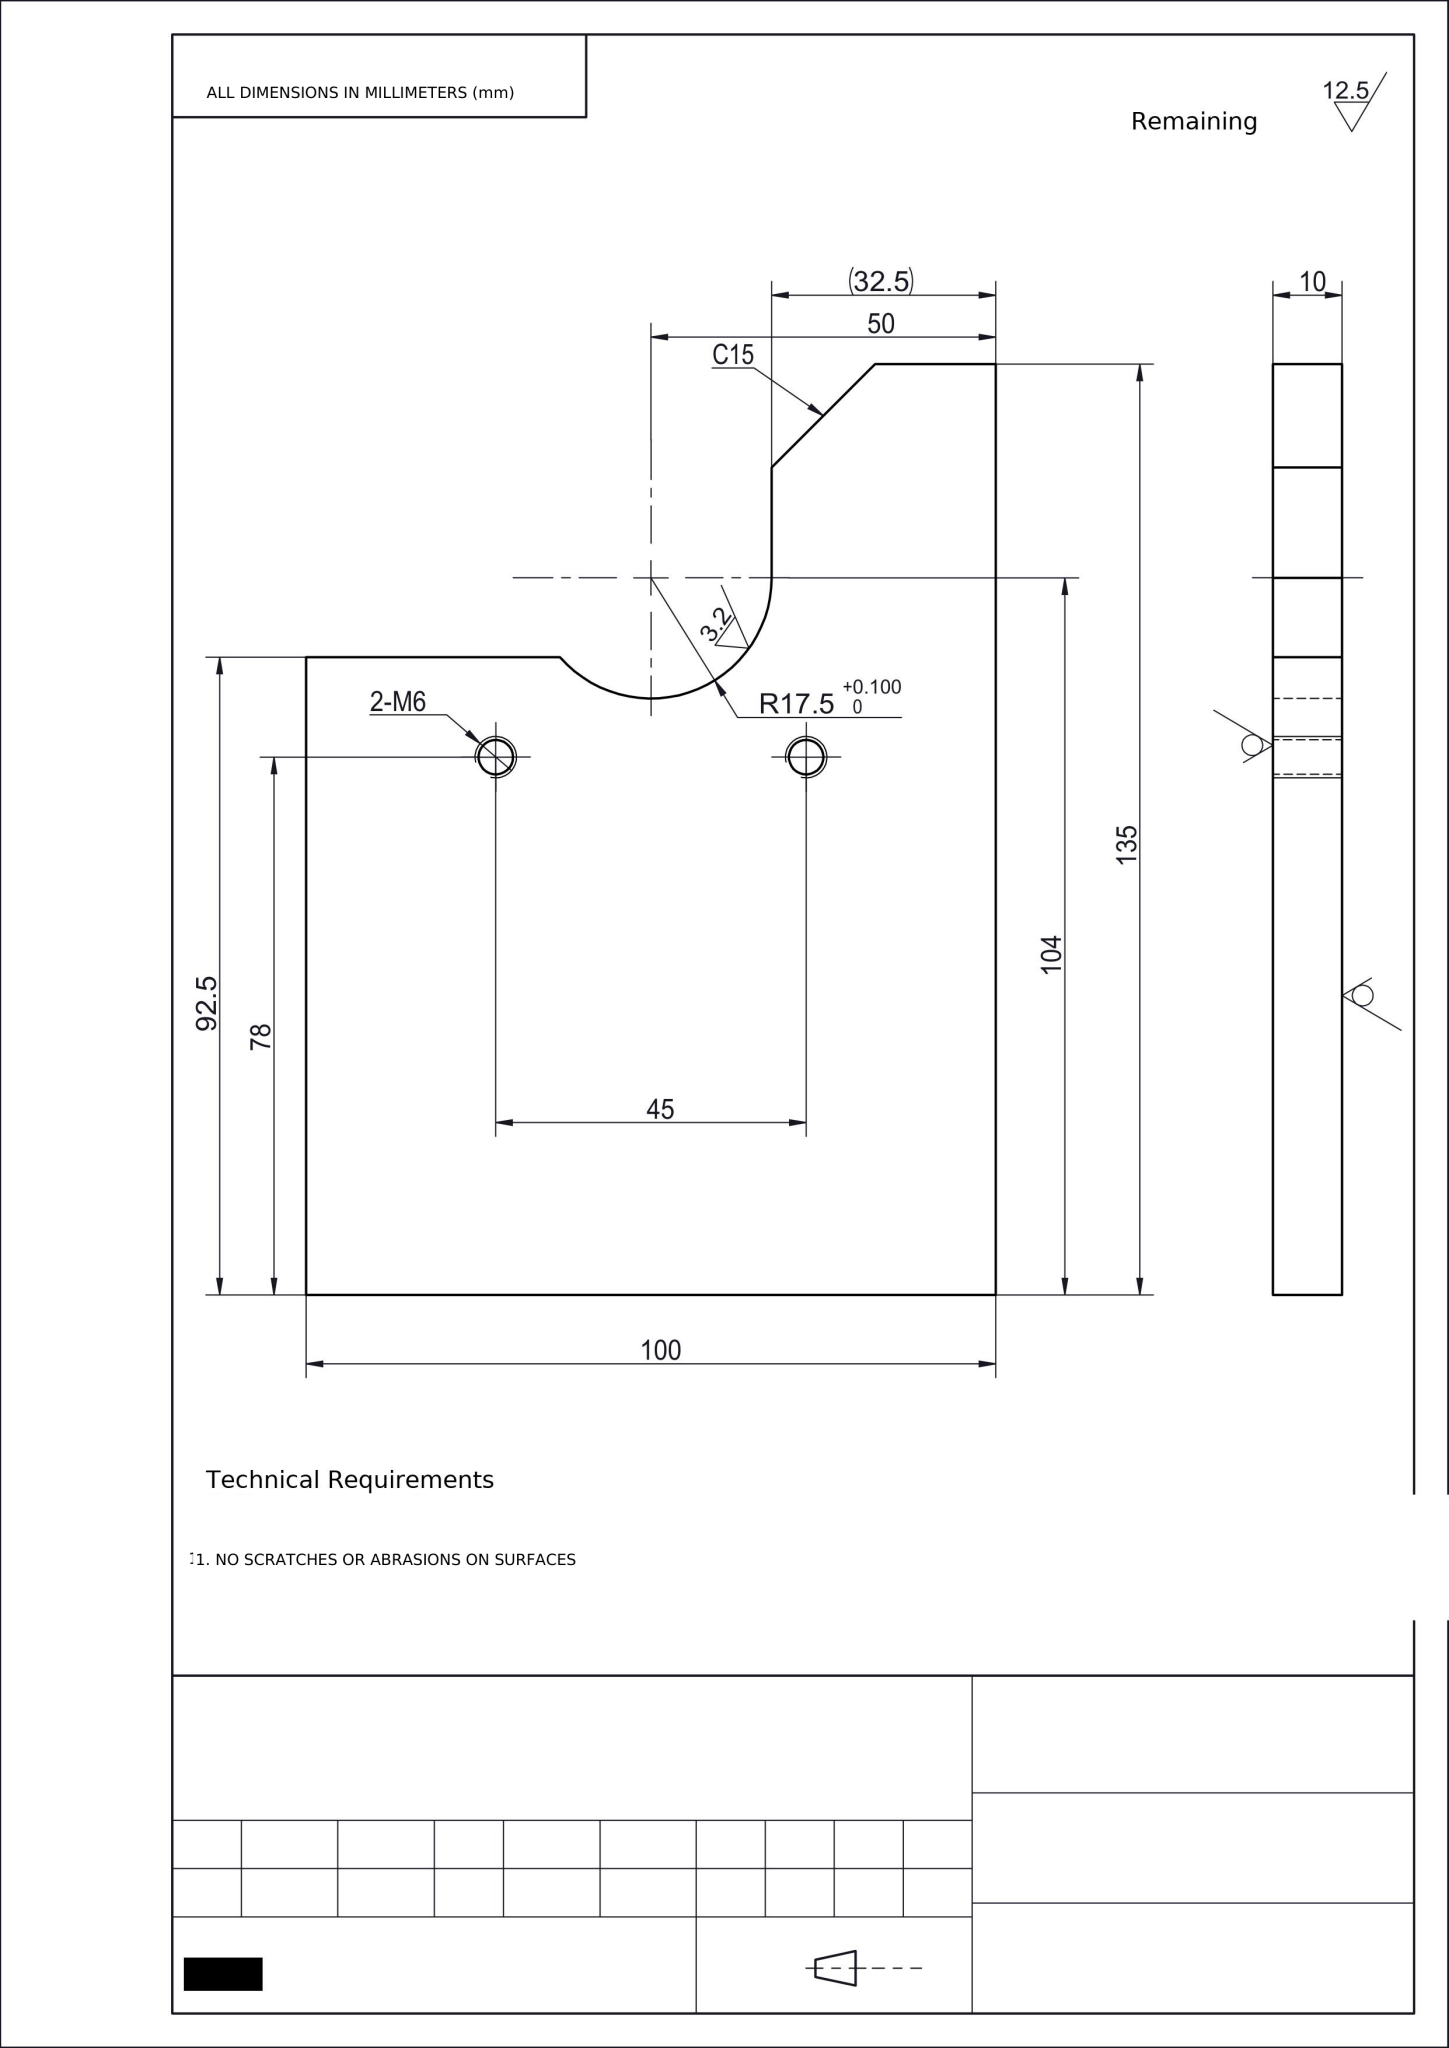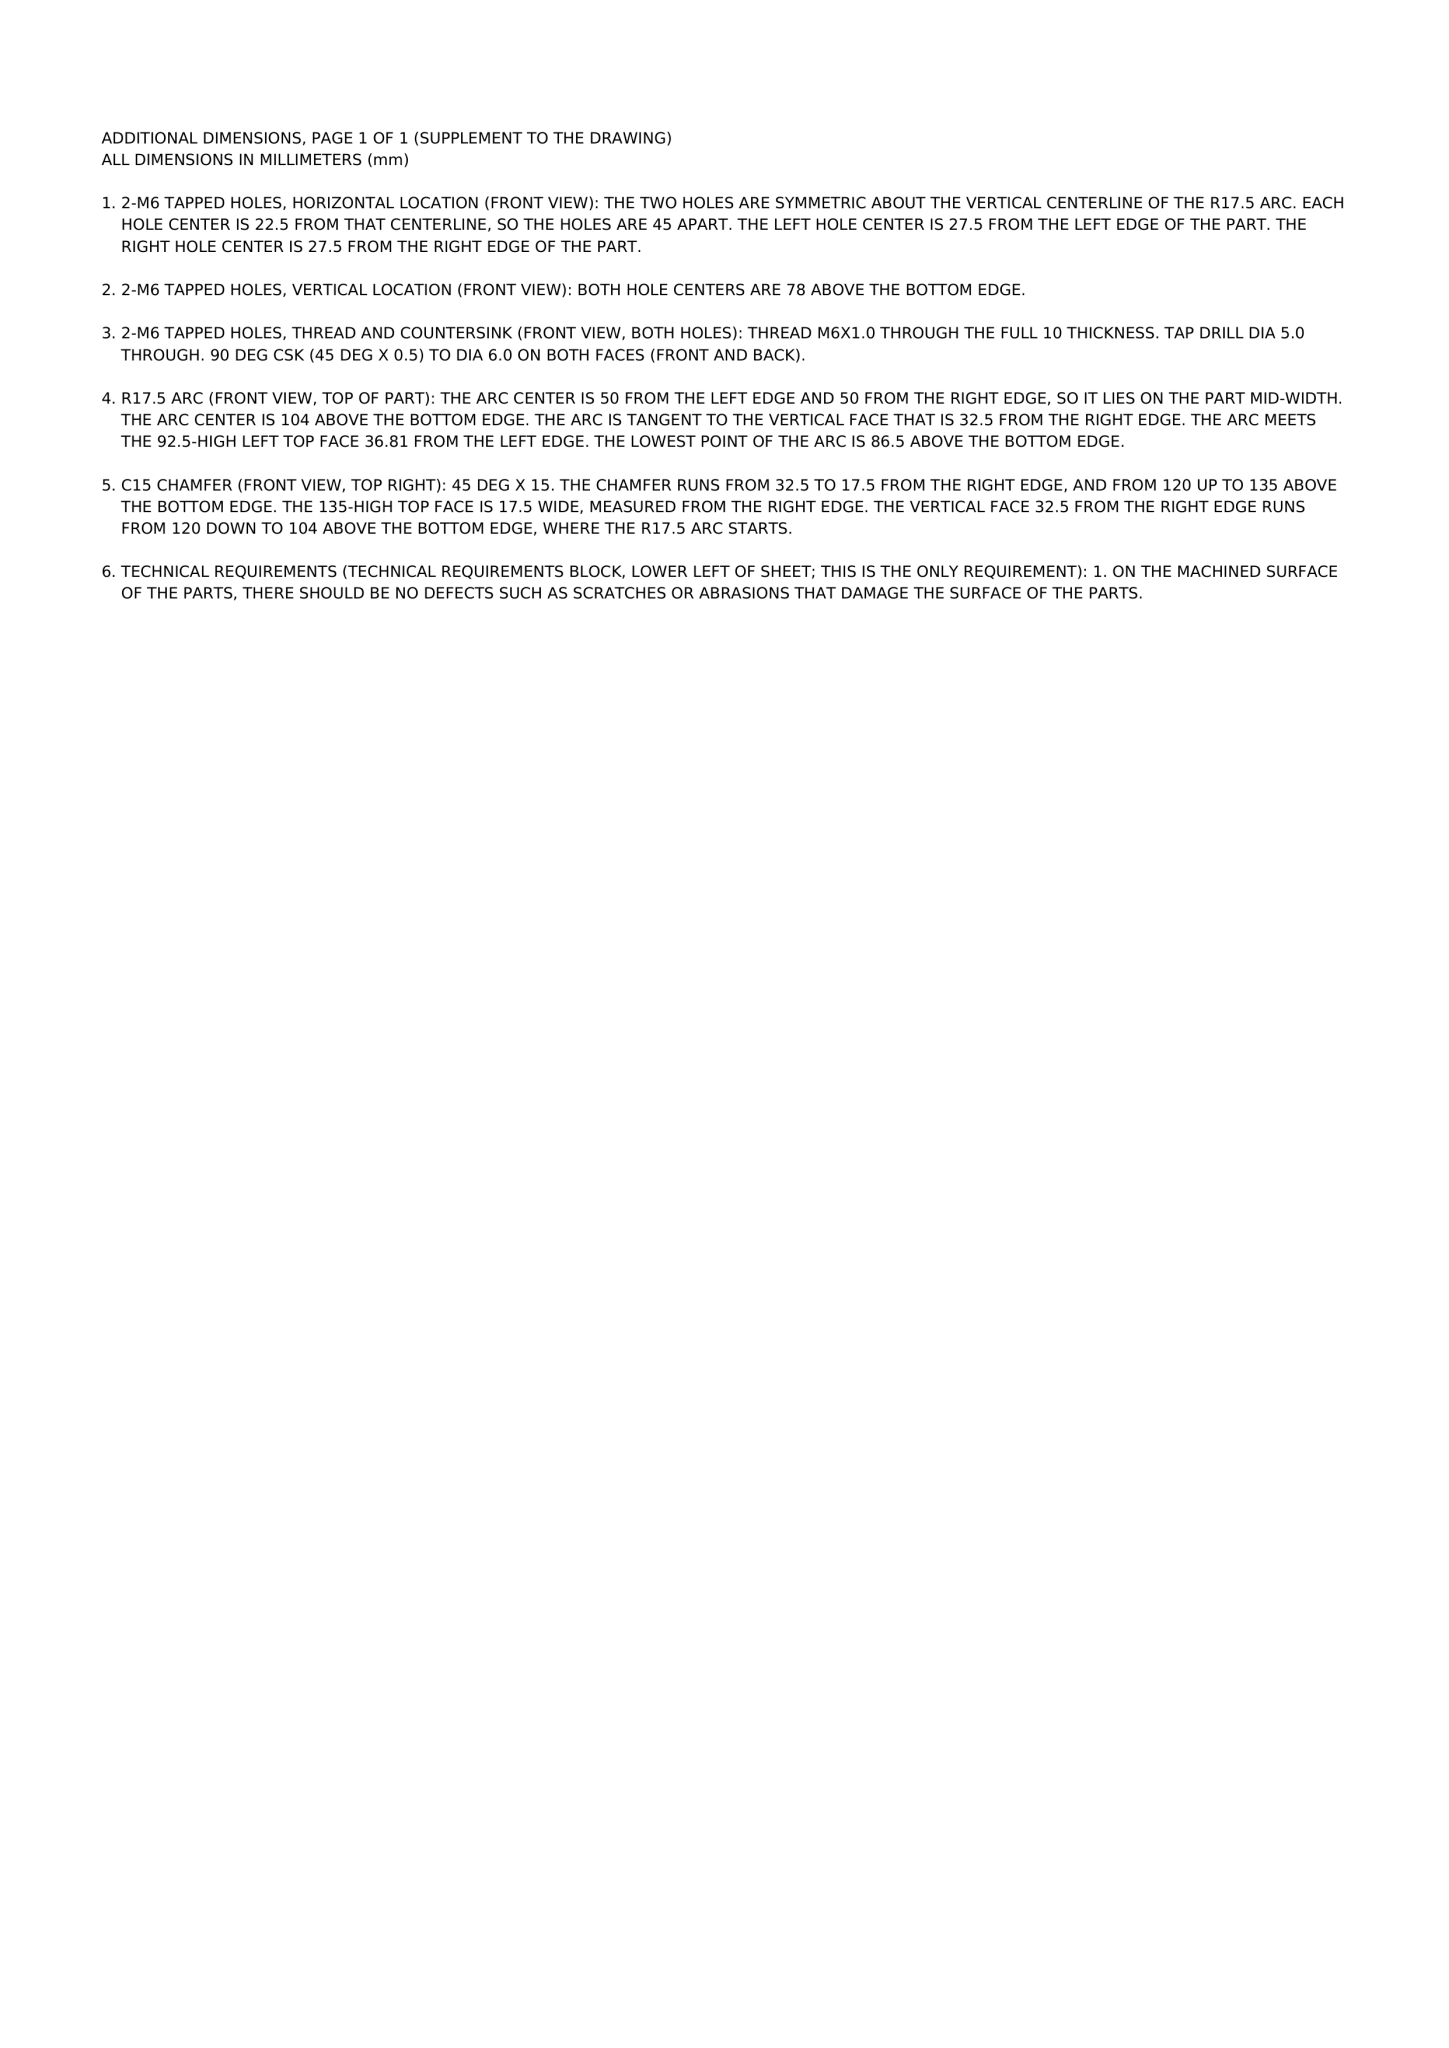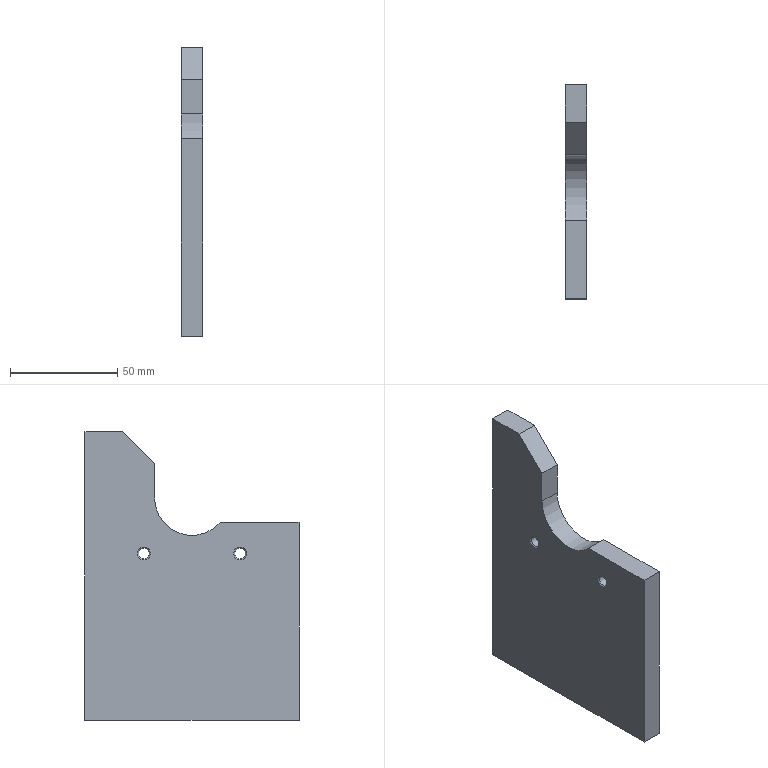Part | NX | mm | 1 solid | 16 faces | box 10 x 100 x 135 mm | volume 103845 mm3 | plane 9 | cone 4 | cylinder 3 | commonest cylinder face diameters 5 x2 35 x1
STEP:
#1=CARTESIAN_POINT('',(0.,0.,0.));
#2=DIRECTION('',(0.,0.,1.));
#3=DIRECTION('',(1.,0.,0.));
#4=AXIS2_PLACEMENT_3D('',#1,#2,#3);
#5=(LENGTH_UNIT()NAMED_UNIT(*)SI_UNIT(.MILLI.,.METRE.));
#6=UNCERTAINTY_MEASURE_WITH_UNIT(LENGTH_MEASURE(0.00002),#5,'','');
#7=(NAMED_UNIT(*)PLANE_ANGLE_UNIT()SI_UNIT($,.RADIAN.));
#8=PLANE_ANGLE_MEASURE_WITH_UNIT(PLANE_ANGLE_MEASURE(0.01745),#7);
#9=DIMENSIONAL_EXPONENTS(0.,0.,0.,0.,0.,0.,0.);
#10=(CONVERSION_BASED_UNIT('',#8)NAMED_UNIT(#9)PLANE_ANGLE_UNIT());
#11=(NAMED_UNIT(*)SI_UNIT($,.STERADIAN.)SOLID_ANGLE_UNIT());
#12=(GEOMETRIC_REPRESENTATION_CONTEXT(3)GLOBAL_UNCERTAINTY_ASSIGNED_CONTEXT((#6))GLOBAL_UNIT_ASSIGNED_CONTEXT((#5,#10,#11))REPRESENTATION_CONTEXT('',''));
#13=SHAPE_REPRESENTATION('',(#4),#12);
#14=CARTESIAN_POINT('',(0.,-50.,92.5));
#15=VERTEX_POINT('',#14);
#16=CARTESIAN_POINT('',(0.,-50.,0.));
#17=VERTEX_POINT('',#16);
#18=CARTESIAN_POINT('',(0.,-50.,92.5));
#19=DIRECTION('',(0.,0.,-1.));
#20=VECTOR('',#19,1.);
#21=LINE('',#18,#20);
#22=EDGE_CURVE('',#15,#17,#21,.T.);
#23=ORIENTED_EDGE('',*,*,#22,.T.);
#24=CARTESIAN_POINT('',(10.,-50.,0.));
#25=VERTEX_POINT('',#24);
#26=CARTESIAN_POINT('',(10.,-50.,0.));
#27=DIRECTION('',(-1.,0.,0.));
#28=VECTOR('',#27,1.);
#29=LINE('',#26,#28);
#30=EDGE_CURVE('',#25,#17,#29,.T.);
#31=ORIENTED_EDGE('',*,*,#30,.F.);
#32=CARTESIAN_POINT('',(10.,-50.,92.5));
#33=VERTEX_POINT('',#32);
#34=CARTESIAN_POINT('',(10.,-50.,92.5));
#35=DIRECTION('',(0.,0.,-1.));
#36=VECTOR('',#35,1.);
#37=LINE('',#34,#36);
#38=EDGE_CURVE('',#33,#25,#37,.T.);
#39=ORIENTED_EDGE('',*,*,#38,.F.);
#40=CARTESIAN_POINT('',(10.,-50.,92.5));
#41=DIRECTION('',(-1.,0.,0.));
#42=VECTOR('',#41,1.);
#43=LINE('',#40,#42);
#44=EDGE_CURVE('',#33,#15,#43,.T.);
#45=ORIENTED_EDGE('',*,*,#44,.T.);
#46=EDGE_LOOP('',(#23,#31,#39,#45));
#47=FACE_OUTER_BOUND('',#46,.T.);
#48=CARTESIAN_POINT('',(10.,-50.,92.5));
#49=DIRECTION('',(0.,1.,0.));
#50=DIRECTION('',(0.,0.,1.));
#51=AXIS2_PLACEMENT_3D('',#48,#49,#50);
#52=PLANE('',#51);
#53=ADVANCED_FACE('',(#47),#52,.F.);
#54=CARTESIAN_POINT('',(0.,50.,0.));
#55=VERTEX_POINT('',#54);
#56=CARTESIAN_POINT('',(0.,-50.,0.));
#57=DIRECTION('',(0.,1.,0.));
#58=VECTOR('',#57,1.);
#59=LINE('',#56,#58);
#60=EDGE_CURVE('',#17,#55,#59,.T.);
#61=ORIENTED_EDGE('',*,*,#60,.T.);
#62=CARTESIAN_POINT('',(10.,50.,0.));
#63=VERTEX_POINT('',#62);
#64=CARTESIAN_POINT('',(10.,50.,0.));
#65=DIRECTION('',(-1.,0.,0.));
#66=VECTOR('',#65,1.);
#67=LINE('',#64,#66);
#68=EDGE_CURVE('',#63,#55,#67,.T.);
#69=ORIENTED_EDGE('',*,*,#68,.F.);
#70=CARTESIAN_POINT('',(10.,-50.,0.));
#71=DIRECTION('',(0.,1.,0.));
#72=VECTOR('',#71,1.);
#73=LINE('',#70,#72);
#74=EDGE_CURVE('',#25,#63,#73,.T.);
#75=ORIENTED_EDGE('',*,*,#74,.F.);
#76=ORIENTED_EDGE('',*,*,#30,.T.);
#77=EDGE_LOOP('',(#61,#69,#75,#76));
#78=FACE_OUTER_BOUND('',#77,.T.);
#79=CARTESIAN_POINT('',(10.,-50.,0.));
#80=DIRECTION('',(0.,0.,1.));
#81=DIRECTION('',(1.,0.,0.));
#82=AXIS2_PLACEMENT_3D('',#79,#80,#81);
#83=PLANE('',#82);
#84=ADVANCED_FACE('',(#78),#83,.F.);
#85=CARTESIAN_POINT('',(0.,50.,135.));
#86=VERTEX_POINT('',#85);
#87=CARTESIAN_POINT('',(0.,50.,0.));
#88=DIRECTION('',(0.,0.,1.));
#89=VECTOR('',#88,1.);
#90=LINE('',#87,#89);
#91=EDGE_CURVE('',#55,#86,#90,.T.);
#92=ORIENTED_EDGE('',*,*,#91,.T.);
#93=CARTESIAN_POINT('',(10.,50.,135.));
#94=VERTEX_POINT('',#93);
#95=CARTESIAN_POINT('',(10.,50.,135.));
#96=DIRECTION('',(-1.,0.,0.));
#97=VECTOR('',#96,1.);
#98=LINE('',#95,#97);
#99=EDGE_CURVE('',#94,#86,#98,.T.);
#100=ORIENTED_EDGE('',*,*,#99,.F.);
#101=CARTESIAN_POINT('',(10.,50.,0.));
#102=DIRECTION('',(0.,0.,1.));
#103=VECTOR('',#102,1.);
#104=LINE('',#101,#103);
#105=EDGE_CURVE('',#63,#94,#104,.T.);
#106=ORIENTED_EDGE('',*,*,#105,.F.);
#107=ORIENTED_EDGE('',*,*,#68,.T.);
#108=EDGE_LOOP('',(#92,#100,#106,#107));
#109=FACE_OUTER_BOUND('',#108,.T.);
#110=CARTESIAN_POINT('',(10.,50.,0.));
#111=DIRECTION('',(0.,-1.,0.));
#112=DIRECTION('',(0.,0.,-1.));
#113=AXIS2_PLACEMENT_3D('',#110,#111,#112);
#114=PLANE('',#113);
#115=ADVANCED_FACE('',(#109),#114,.F.);
#116=CARTESIAN_POINT('',(0.,32.5,135.));
#117=VERTEX_POINT('',#116);
#118=CARTESIAN_POINT('',(0.,50.,135.));
#119=DIRECTION('',(0.,-1.,0.));
#120=VECTOR('',#119,1.);
#121=LINE('',#118,#120);
#122=EDGE_CURVE('',#86,#117,#121,.T.);
#123=ORIENTED_EDGE('',*,*,#122,.T.);
#124=CARTESIAN_POINT('',(10.,32.5,135.));
#125=VERTEX_POINT('',#124);
#126=CARTESIAN_POINT('',(10.,32.5,135.));
#127=DIRECTION('',(1.,0.,0.));
#128=VECTOR('',#127,1.);
#129=LINE('',#126,#128);
#130=EDGE_CURVE('',#117,#125,#129,.T.);
#131=ORIENTED_EDGE('',*,*,#130,.T.);
#132=CARTESIAN_POINT('',(10.,50.,135.));
#133=DIRECTION('',(0.,-1.,0.));
#134=VECTOR('',#133,1.);
#135=LINE('',#132,#134);
#136=EDGE_CURVE('',#94,#125,#135,.T.);
#137=ORIENTED_EDGE('',*,*,#136,.F.);
#138=ORIENTED_EDGE('',*,*,#99,.T.);
#139=EDGE_LOOP('',(#123,#131,#137,#138));
#140=FACE_OUTER_BOUND('',#139,.T.);
#141=CARTESIAN_POINT('',(10.,50.,135.));
#142=DIRECTION('',(0.,0.,-1.));
#143=DIRECTION('',(-1.,0.,0.));
#144=AXIS2_PLACEMENT_3D('',#141,#142,#143);
#145=PLANE('',#144);
#146=ADVANCED_FACE('',(#140),#145,.F.);
#147=CARTESIAN_POINT('',(10.,17.5,120.));
#148=VERTEX_POINT('',#147);
#149=CARTESIAN_POINT('',(10.,17.5,104.));
#150=VERTEX_POINT('',#149);
#151=CARTESIAN_POINT('',(10.,17.5,135.));
#152=DIRECTION('',(0.,0.,-1.));
#153=VECTOR('',#152,1.);
#154=LINE('',#151,#153);
#155=EDGE_CURVE('',#148,#150,#154,.T.);
#156=ORIENTED_EDGE('',*,*,#155,.F.);
#157=CARTESIAN_POINT('',(0.,17.5,120.));
#158=VERTEX_POINT('',#157);
#159=CARTESIAN_POINT('',(10.,17.5,120.));
#160=DIRECTION('',(-1.,0.,0.));
#161=VECTOR('',#160,1.);
#162=LINE('',#159,#161);
#163=EDGE_CURVE('',#148,#158,#162,.T.);
#164=ORIENTED_EDGE('',*,*,#163,.T.);
#165=CARTESIAN_POINT('',(0.,17.5,104.));
#166=VERTEX_POINT('',#165);
#167=CARTESIAN_POINT('',(0.,17.5,135.));
#168=DIRECTION('',(0.,0.,-1.));
#169=VECTOR('',#168,1.);
#170=LINE('',#167,#169);
#171=EDGE_CURVE('',#158,#166,#170,.T.);
#172=ORIENTED_EDGE('',*,*,#171,.T.);
#173=CARTESIAN_POINT('',(10.,17.5,104.));
#174=DIRECTION('',(-1.,0.,0.));
#175=VECTOR('',#174,1.);
#176=LINE('',#173,#175);
#177=EDGE_CURVE('',#150,#166,#176,.T.);
#178=ORIENTED_EDGE('',*,*,#177,.F.);
#179=EDGE_LOOP('',(#156,#164,#172,#178));
#180=FACE_OUTER_BOUND('',#179,.T.);
#181=CARTESIAN_POINT('',(10.,17.5,135.));
#182=DIRECTION('',(0.,1.,0.));
#183=DIRECTION('',(0.,0.,1.));
#184=AXIS2_PLACEMENT_3D('',#181,#182,#183);
#185=PLANE('',#184);
#186=ADVANCED_FACE('',(#180),#185,.F.);
#187=CARTESIAN_POINT('',(0.,-13.191,92.5));
#188=VERTEX_POINT('',#187);
#189=CARTESIAN_POINT('',(0.,0.,104.));
#190=DIRECTION('',(-1.,0.,0.));
#191=DIRECTION('',(0.,1.,0.));
#192=AXIS2_PLACEMENT_3D('',#189,#190,#191);
#193=CIRCLE('',#192,17.5);
#194=EDGE_CURVE('',#166,#188,#193,.T.);
#195=ORIENTED_EDGE('',*,*,#194,.T.);
#196=CARTESIAN_POINT('',(10.,-13.191,92.5));
#197=VERTEX_POINT('',#196);
#198=CARTESIAN_POINT('',(10.,-13.191,92.5));
#199=DIRECTION('',(-1.,0.,0.));
#200=VECTOR('',#199,1.);
#201=LINE('',#198,#200);
#202=EDGE_CURVE('',#197,#188,#201,.T.);
#203=ORIENTED_EDGE('',*,*,#202,.F.);
#204=CARTESIAN_POINT('',(10.,0.,104.));
#205=DIRECTION('',(-1.,0.,0.));
#206=DIRECTION('',(0.,1.,0.));
#207=AXIS2_PLACEMENT_3D('',#204,#205,#206);
#208=CIRCLE('',#207,17.5);
#209=EDGE_CURVE('',#150,#197,#208,.T.);
#210=ORIENTED_EDGE('',*,*,#209,.F.);
#211=ORIENTED_EDGE('',*,*,#177,.T.);
#212=EDGE_LOOP('',(#195,#203,#210,#211));
#213=FACE_OUTER_BOUND('',#212,.T.);
#214=CARTESIAN_POINT('',(10.,0.,104.));
#215=DIRECTION('',(-1.,0.,0.));
#216=DIRECTION('',(0.,0.,1.));
#217=AXIS2_PLACEMENT_3D('',#214,#215,#216);
#218=CYLINDRICAL_SURFACE('',#217,17.5);
#219=ADVANCED_FACE('',(#213),#218,.F.);
#220=CARTESIAN_POINT('',(0.,-13.191,92.5));
#221=DIRECTION('',(0.,-1.,0.));
#222=VECTOR('',#221,1.);
#223=LINE('',#220,#222);
#224=EDGE_CURVE('',#188,#15,#223,.T.);
#225=ORIENTED_EDGE('',*,*,#224,.T.);
#226=ORIENTED_EDGE('',*,*,#44,.F.);
#227=CARTESIAN_POINT('',(10.,-13.191,92.5));
#228=DIRECTION('',(0.,-1.,0.));
#229=VECTOR('',#228,1.);
#230=LINE('',#227,#229);
#231=EDGE_CURVE('',#197,#33,#230,.T.);
#232=ORIENTED_EDGE('',*,*,#231,.F.);
#233=ORIENTED_EDGE('',*,*,#202,.T.);
#234=EDGE_LOOP('',(#225,#226,#232,#233));
#235=FACE_OUTER_BOUND('',#234,.T.);
#236=CARTESIAN_POINT('',(10.,-13.191,92.5));
#237=DIRECTION('',(0.,0.,-1.));
#238=DIRECTION('',(-1.,0.,0.));
#239=AXIS2_PLACEMENT_3D('',#236,#237,#238);
#240=PLANE('',#239);
#241=ADVANCED_FACE('',(#235),#240,.F.);
#242=CARTESIAN_POINT('',(10.,-22.5,81.));
#243=VERTEX_POINT('',#242);
#244=CARTESIAN_POINT('',(10.,-22.5,78.));
#245=DIRECTION('',(-1.,0.,0.));
#246=DIRECTION('',(0.,0.,1.));
#247=AXIS2_PLACEMENT_3D('',#244,#245,#246);
#248=CIRCLE('',#247,3.);
#249=EDGE_CURVE('',#243,#243,#248,.T.);
#250=ORIENTED_EDGE('',*,*,#249,.T.);
#251=EDGE_LOOP('',(#250));
#252=FACE_BOUND('',#251,.T.);
#253=CARTESIAN_POINT('',(10.,22.5,81.));
#254=VERTEX_POINT('',#253);
#255=CARTESIAN_POINT('',(10.,22.5,78.));
#256=DIRECTION('',(-1.,0.,0.));
#257=DIRECTION('',(0.,0.,1.));
#258=AXIS2_PLACEMENT_3D('',#255,#256,#257);
#259=CIRCLE('',#258,3.);
#260=EDGE_CURVE('',#254,#254,#259,.T.);
#261=ORIENTED_EDGE('',*,*,#260,.T.);
#262=EDGE_LOOP('',(#261));
#263=FACE_BOUND('',#262,.T.);
#264=ORIENTED_EDGE('',*,*,#136,.T.);
#265=CARTESIAN_POINT('',(10.,17.5,120.));
#266=DIRECTION('',(0.,-0.7071,-0.7071));
#267=VECTOR('',#266,1.);
#268=LINE('',#265,#267);
#269=EDGE_CURVE('',#125,#148,#268,.T.);
#270=ORIENTED_EDGE('',*,*,#269,.T.);
#271=ORIENTED_EDGE('',*,*,#155,.T.);
#272=ORIENTED_EDGE('',*,*,#209,.T.);
#273=ORIENTED_EDGE('',*,*,#231,.T.);
#274=ORIENTED_EDGE('',*,*,#38,.T.);
#275=ORIENTED_EDGE('',*,*,#74,.T.);
#276=ORIENTED_EDGE('',*,*,#105,.T.);
#277=EDGE_LOOP('',(#264,#270,#271,#272,#273,#274,#275,#276));
#278=FACE_BOUND('',#277,.T.);
#279=CARTESIAN_POINT('',(10.,0.,104.));
#280=DIRECTION('',(-1.,0.,0.));
#281=DIRECTION('',(0.,0.,1.));
#282=AXIS2_PLACEMENT_3D('',#279,#280,#281);
#283=PLANE('',#282);
#284=ADVANCED_FACE('',(#252,#263,#278),#283,.F.);
#285=CARTESIAN_POINT('',(0.,-22.5,81.));
#286=VERTEX_POINT('',#285);
#287=CARTESIAN_POINT('',(0.,-22.5,78.));
#288=DIRECTION('',(-1.,0.,0.));
#289=DIRECTION('',(0.,0.,1.));
#290=AXIS2_PLACEMENT_3D('',#287,#288,#289);
#291=CIRCLE('',#290,3.);
#292=EDGE_CURVE('',#286,#286,#291,.T.);
#293=ORIENTED_EDGE('',*,*,#292,.F.);
#294=EDGE_LOOP('',(#293));
#295=FACE_BOUND('',#294,.T.);
#296=CARTESIAN_POINT('',(0.,22.5,81.));
#297=VERTEX_POINT('',#296);
#298=CARTESIAN_POINT('',(0.,22.5,78.));
#299=DIRECTION('',(-1.,0.,0.));
#300=DIRECTION('',(0.,0.,1.));
#301=AXIS2_PLACEMENT_3D('',#298,#299,#300);
#302=CIRCLE('',#301,3.);
#303=EDGE_CURVE('',#297,#297,#302,.T.);
#304=ORIENTED_EDGE('',*,*,#303,.F.);
#305=EDGE_LOOP('',(#304));
#306=FACE_BOUND('',#305,.T.);
#307=ORIENTED_EDGE('',*,*,#171,.F.);
#308=CARTESIAN_POINT('',(0.,0.75,103.25));
#309=DIRECTION('',(0.,0.7071,0.7071));
#310=VECTOR('',#309,1.);
#311=LINE('',#308,#310);
#312=EDGE_CURVE('',#158,#117,#311,.T.);
#313=ORIENTED_EDGE('',*,*,#312,.T.);
#314=ORIENTED_EDGE('',*,*,#122,.F.);
#315=ORIENTED_EDGE('',*,*,#91,.F.);
#316=ORIENTED_EDGE('',*,*,#60,.F.);
#317=ORIENTED_EDGE('',*,*,#22,.F.);
#318=ORIENTED_EDGE('',*,*,#224,.F.);
#319=ORIENTED_EDGE('',*,*,#194,.F.);
#320=EDGE_LOOP('',(#307,#313,#314,#315,#316,#317,#318,#319));
#321=FACE_BOUND('',#320,.T.);
#322=CARTESIAN_POINT('',(0.,0.,104.));
#323=DIRECTION('',(-1.,0.,0.));
#324=DIRECTION('',(0.,0.,1.));
#325=AXIS2_PLACEMENT_3D('',#322,#323,#324);
#326=PLANE('',#325);
#327=ADVANCED_FACE('',(#295,#306,#321),#326,.T.);
#328=CARTESIAN_POINT('',(9.5,22.5,75.5));
#329=VERTEX_POINT('',#328);
#330=CARTESIAN_POINT('',(9.5,22.5,78.));
#331=DIRECTION('',(1.,0.,0.));
#332=DIRECTION('',(0.,0.,-1.));
#333=AXIS2_PLACEMENT_3D('',#330,#331,#332);
#334=CIRCLE('',#333,2.5);
#335=EDGE_CURVE('',#329,#329,#334,.T.);
#336=ORIENTED_EDGE('',*,*,#335,.T.);
#337=EDGE_LOOP('',(#336));
#338=FACE_BOUND('',#337,.T.);
#339=CARTESIAN_POINT('',(0.5,22.5,80.5));
#340=VERTEX_POINT('',#339);
#341=CARTESIAN_POINT('',(0.5,22.5,78.));
#342=DIRECTION('',(-1.,0.,0.));
#343=DIRECTION('',(0.,0.,1.));
#344=AXIS2_PLACEMENT_3D('',#341,#342,#343);
#345=CIRCLE('',#344,2.5);
#346=EDGE_CURVE('',#340,#340,#345,.T.);
#347=ORIENTED_EDGE('',*,*,#346,.T.);
#348=EDGE_LOOP('',(#347));
#349=FACE_BOUND('',#348,.T.);
#350=CARTESIAN_POINT('',(0.,22.5,78.));
#351=DIRECTION('',(1.,0.,0.));
#352=DIRECTION('',(0.,0.,-1.));
#353=AXIS2_PLACEMENT_3D('',#350,#351,#352);
#354=CYLINDRICAL_SURFACE('',#353,2.5);
#355=ADVANCED_FACE('',(#338,#349),#354,.F.);
#356=ORIENTED_EDGE('',*,*,#303,.T.);
#357=EDGE_LOOP('',(#356));
#358=FACE_BOUND('',#357,.T.);
#359=ORIENTED_EDGE('',*,*,#346,.F.);
#360=EDGE_LOOP('',(#359));
#361=FACE_BOUND('',#360,.T.);
#362=CARTESIAN_POINT('',(3.,22.5,78.));
#363=DIRECTION('',(-1.,0.,0.));
#364=DIRECTION('',(-0.,-1.,0.));
#365=AXIS2_PLACEMENT_3D('',#362,#363,#364);
#366=CONICAL_SURFACE('',#365,0.,45.);
#367=ADVANCED_FACE('',(#358,#361),#366,.F.);
#368=ORIENTED_EDGE('',*,*,#260,.F.);
#369=EDGE_LOOP('',(#368));
#370=FACE_BOUND('',#369,.T.);
#371=ORIENTED_EDGE('',*,*,#335,.F.);
#372=EDGE_LOOP('',(#371));
#373=FACE_BOUND('',#372,.T.);
#374=CARTESIAN_POINT('',(7.,22.5,78.));
#375=DIRECTION('',(1.,0.,0.));
#376=DIRECTION('',(-0.,1.,0.));
#377=AXIS2_PLACEMENT_3D('',#374,#375,#376);
#378=CONICAL_SURFACE('',#377,0.,45.);
#379=ADVANCED_FACE('',(#370,#373),#378,.F.);
#380=CARTESIAN_POINT('',(9.5,-22.5,75.5));
#381=VERTEX_POINT('',#380);
#382=CARTESIAN_POINT('',(9.5,-22.5,78.));
#383=DIRECTION('',(1.,0.,0.));
#384=DIRECTION('',(0.,0.,-1.));
#385=AXIS2_PLACEMENT_3D('',#382,#383,#384);
#386=CIRCLE('',#385,2.5);
#387=EDGE_CURVE('',#381,#381,#386,.T.);
#388=ORIENTED_EDGE('',*,*,#387,.T.);
#389=EDGE_LOOP('',(#388));
#390=FACE_BOUND('',#389,.T.);
#391=CARTESIAN_POINT('',(0.5,-22.5,80.5));
#392=VERTEX_POINT('',#391);
#393=CARTESIAN_POINT('',(0.5,-22.5,78.));
#394=DIRECTION('',(-1.,0.,0.));
#395=DIRECTION('',(0.,0.,1.));
#396=AXIS2_PLACEMENT_3D('',#393,#394,#395);
#397=CIRCLE('',#396,2.5);
#398=EDGE_CURVE('',#392,#392,#397,.T.);
#399=ORIENTED_EDGE('',*,*,#398,.T.);
#400=EDGE_LOOP('',(#399));
#401=FACE_BOUND('',#400,.T.);
#402=CARTESIAN_POINT('',(0.,-22.5,78.));
#403=DIRECTION('',(1.,0.,0.));
#404=DIRECTION('',(0.,0.,-1.));
#405=AXIS2_PLACEMENT_3D('',#402,#403,#404);
#406=CYLINDRICAL_SURFACE('',#405,2.5);
#407=ADVANCED_FACE('',(#390,#401),#406,.F.);
#408=ORIENTED_EDGE('',*,*,#292,.T.);
#409=EDGE_LOOP('',(#408));
#410=FACE_BOUND('',#409,.T.);
#411=ORIENTED_EDGE('',*,*,#398,.F.);
#412=EDGE_LOOP('',(#411));
#413=FACE_BOUND('',#412,.T.);
#414=CARTESIAN_POINT('',(3.,-22.5,78.));
#415=DIRECTION('',(-1.,0.,0.));
#416=DIRECTION('',(-0.,-1.,0.));
#417=AXIS2_PLACEMENT_3D('',#414,#415,#416);
#418=CONICAL_SURFACE('',#417,0.,45.);
#419=ADVANCED_FACE('',(#410,#413),#418,.F.);
#420=ORIENTED_EDGE('',*,*,#249,.F.);
#421=EDGE_LOOP('',(#420));
#422=FACE_BOUND('',#421,.T.);
#423=ORIENTED_EDGE('',*,*,#387,.F.);
#424=EDGE_LOOP('',(#423));
#425=FACE_BOUND('',#424,.T.);
#426=CARTESIAN_POINT('',(7.,-22.5,78.));
#427=DIRECTION('',(1.,0.,0.));
#428=DIRECTION('',(-0.,1.,0.));
#429=AXIS2_PLACEMENT_3D('',#426,#427,#428);
#430=CONICAL_SURFACE('',#429,0.,45.);
#431=ADVANCED_FACE('',(#422,#425),#430,.F.);
#432=ORIENTED_EDGE('',*,*,#269,.F.);
#433=ORIENTED_EDGE('',*,*,#130,.F.);
#434=ORIENTED_EDGE('',*,*,#312,.F.);
#435=ORIENTED_EDGE('',*,*,#163,.F.);
#436=EDGE_LOOP('',(#432,#433,#434,#435));
#437=FACE_OUTER_BOUND('',#436,.T.);
#438=CARTESIAN_POINT('',(10.,17.5,120.));
#439=DIRECTION('',(0.,0.7071,-0.7071));
#440=DIRECTION('',(-1.,0.,0.));
#441=AXIS2_PLACEMENT_3D('',#438,#439,#440);
#442=PLANE('',#441);
#443=ADVANCED_FACE('',(#437),#442,.F.);
#444=CLOSED_SHELL('',(#53,#84,#115,#146,#186,#219,#241,#284,#327,#355,#367,#379,#407,#419,#431,#443));
#445=MANIFOLD_SOLID_BREP('',#444);
#446=ADVANCED_BREP_SHAPE_REPRESENTATION('',(#445),#12);
#447=SHAPE_REPRESENTATION_RELATIONSHIP('','',#13,#446);
#448=PRESENTATION_LAYER_ASSIGNMENT('','',(#445));
#449=COLOUR_RGB('',1.,0.6,0.);
#450=FILL_AREA_STYLE_COLOUR('',#449);
#451=FILL_AREA_STYLE('',(#450));
#452=SURFACE_STYLE_FILL_AREA(#451);
#453=SURFACE_SIDE_STYLE('',(#452));
#454=SURFACE_STYLE_USAGE(.BOTH.,#453);
#455=PRESENTATION_STYLE_ASSIGNMENT((#454));
#456=STYLED_ITEM('',(#455),#445);
#457=MECHANICAL_DESIGN_GEOMETRIC_PRESENTATION_REPRESENTATION('',(#456),#12);